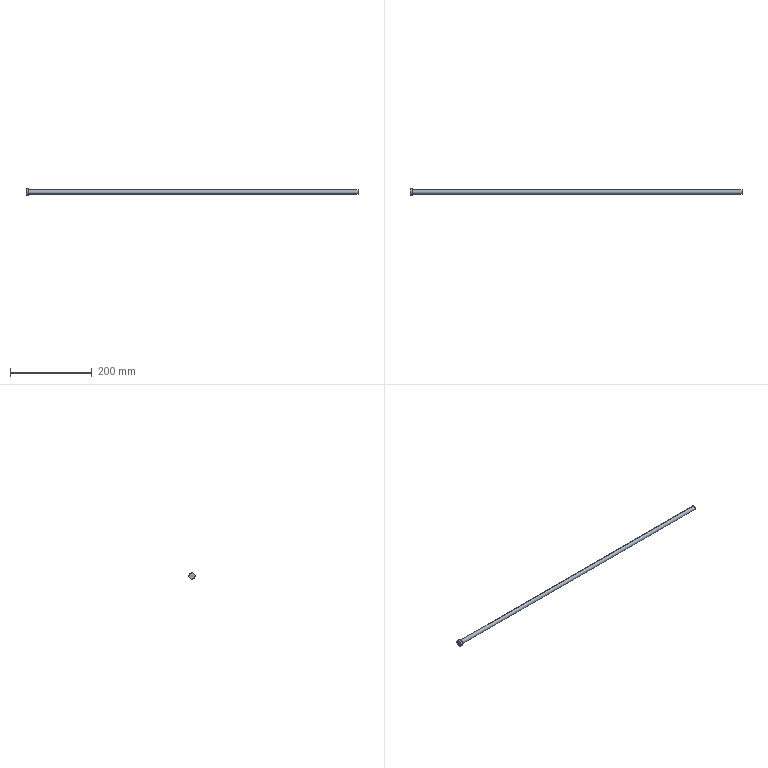Component | SolidWorks | SupportFastAxis-2 | 1 solid | 7 faces | box 811 x 15 x 15 mm | volume 64187 mm3 | cylinder 4 | plane 3 | commonest cylinder face diameters 15 x2 10 x2
build123d program:
from build123d import *

# Parameters (mm, degrees)
SKETCH1_R           = 5
BOSS_EXTRUDE1_DEPTH = 806
SKETCH2_R           = 7.5
BOSS_EXTRUDE2_DEPTH = 5


with BuildPart() as part:
    # Sketch1 → Boss-Extrude1 (new body)
    with BuildSketch(Plane.XY):
        with Locations((90, -65)):
            Circle(SKETCH1_R)
    extrude(amount=-BOSS_EXTRUDE1_DEPTH)

    # Sketch2 → Boss-Extrude2 (add)
    with BuildSketch(Plane.XY):
        with Locations((90, -65)):
            Circle(SKETCH2_R)
    extrude(amount=BOSS_EXTRUDE2_DEPTH)


solid = part.part

# Placed as in the assembly
solid = solid.moved(Location((-400, 155, -25), (0, -90, 0)))
STEP:
#1=COLOUR_RGB('',0.7922,0.8196,0.9333);
#2=FILL_AREA_STYLE_COLOUR('',#1);
#3=FILL_AREA_STYLE('',(#2));
#4=SURFACE_STYLE_FILL_AREA(#3);
#5=SURFACE_SIDE_STYLE('',(#4));
#6=SURFACE_STYLE_USAGE(.BOTH.,#5);
#7=PRESENTATION_STYLE_ASSIGNMENT((#6));
#8=CARTESIAN_POINT('',(-15.945,3.448,2.279));
#9=VERTEX_POINT('',#8);
#10=CARTESIAN_POINT('',(-15.945,3.638,2.839));
#11=VERTEX_POINT('',#10);
#12=CARTESIAN_POINT('',(-15.945,3.543,2.559));
#13=DIRECTION('',(-1.,0.,0.));
#14=DIRECTION('',(0.,-0.3218,-0.9468));
#15=AXIS2_PLACEMENT_3D('',#12,#13,#14);
#16=CIRCLE('',#15,0.2953);
#17=EDGE_CURVE('',#9,#11,#16,.T.);
#18=ORIENTED_EDGE('',*,*,#17,.F.);
#19=CARTESIAN_POINT('',(-15.748,3.448,2.279));
#20=VERTEX_POINT('',#19);
#21=CARTESIAN_POINT('',(-15.945,3.448,2.279));
#22=DIRECTION('',(1.,0.,0.));
#23=VECTOR('',#22,39.37);
#24=LINE('',#21,#23);
#25=EDGE_CURVE('',#9,#20,#24,.T.);
#26=ORIENTED_EDGE('',*,*,#25,.T.);
#27=CARTESIAN_POINT('',(-15.748,3.638,2.839));
#28=VERTEX_POINT('',#27);
#29=CARTESIAN_POINT('',(-15.748,3.543,2.559));
#30=DIRECTION('',(-1.,0.,0.));
#31=DIRECTION('',(0.,-0.3218,-0.9468));
#32=AXIS2_PLACEMENT_3D('',#29,#30,#31);
#33=CIRCLE('',#32,0.2953);
#34=EDGE_CURVE('',#20,#28,#33,.T.);
#35=ORIENTED_EDGE('',*,*,#34,.T.);
#36=CARTESIAN_POINT('',(-15.945,3.638,2.839));
#37=DIRECTION('',(1.,0.,0.));
#38=VECTOR('',#37,39.37);
#39=LINE('',#36,#38);
#40=EDGE_CURVE('',#11,#28,#39,.T.);
#41=ORIENTED_EDGE('',*,*,#40,.F.);
#42=EDGE_LOOP('',(#18,#26,#35,#41));
#43=FACE_OUTER_BOUND('',#42,.T.);
#44=CARTESIAN_POINT('',(-15.945,3.543,2.559));
#45=DIRECTION('',(1.,0.,0.));
#46=DIRECTION('',(0.,0.3218,0.9468));
#47=AXIS2_PLACEMENT_3D('',#44,#45,#46);
#48=CYLINDRICAL_SURFACE('',#47,0.2953);
#49=ADVANCED_FACE('',(#43),#48,.T.);
#50=CARTESIAN_POINT('',(15.984,3.48,2.373));
#51=VERTEX_POINT('',#50);
#52=CARTESIAN_POINT('',(15.984,3.607,2.745));
#53=VERTEX_POINT('',#52);
#54=CARTESIAN_POINT('',(15.984,3.543,2.559));
#55=DIRECTION('',(-1.,0.,0.));
#56=DIRECTION('',(0.,-0.3218,-0.9468));
#57=AXIS2_PLACEMENT_3D('',#54,#55,#56);
#58=CIRCLE('',#57,0.1969);
#59=EDGE_CURVE('',#51,#53,#58,.T.);
#60=ORIENTED_EDGE('',*,*,#59,.T.);
#61=CARTESIAN_POINT('',(-15.748,3.607,2.745));
#62=VERTEX_POINT('',#61);
#63=CARTESIAN_POINT('',(15.984,3.607,2.745));
#64=DIRECTION('',(-1.,0.,0.));
#65=VECTOR('',#64,39.37);
#66=LINE('',#63,#65);
#67=EDGE_CURVE('',#53,#62,#66,.T.);
#68=ORIENTED_EDGE('',*,*,#67,.T.);
#69=CARTESIAN_POINT('',(-15.748,3.48,2.373));
#70=VERTEX_POINT('',#69);
#71=CARTESIAN_POINT('',(-15.748,3.543,2.559));
#72=DIRECTION('',(-1.,0.,0.));
#73=DIRECTION('',(0.,-0.3218,-0.9468));
#74=AXIS2_PLACEMENT_3D('',#71,#72,#73);
#75=CIRCLE('',#74,0.1969);
#76=EDGE_CURVE('',#70,#62,#75,.T.);
#77=ORIENTED_EDGE('',*,*,#76,.F.);
#78=CARTESIAN_POINT('',(15.984,3.48,2.373));
#79=DIRECTION('',(-1.,0.,0.));
#80=VECTOR('',#79,39.37);
#81=LINE('',#78,#80);
#82=EDGE_CURVE('',#51,#70,#81,.T.);
#83=ORIENTED_EDGE('',*,*,#82,.F.);
#84=EDGE_LOOP('',(#60,#68,#77,#83));
#85=FACE_OUTER_BOUND('',#84,.T.);
#86=CARTESIAN_POINT('',(15.984,3.543,2.559));
#87=DIRECTION('',(-1.,0.,0.));
#88=DIRECTION('',(0.,-0.3218,-0.9468));
#89=AXIS2_PLACEMENT_3D('',#86,#87,#88);
#90=CYLINDRICAL_SURFACE('',#89,0.1969);
#91=ADVANCED_FACE('',(#85),#90,.T.);
#92=ORIENTED_EDGE('',*,*,#67,.F.);
#93=CARTESIAN_POINT('',(15.984,3.543,2.559));
#94=DIRECTION('',(-1.,0.,0.));
#95=DIRECTION('',(0.,-0.3218,-0.9468));
#96=AXIS2_PLACEMENT_3D('',#93,#94,#95);
#97=CIRCLE('',#96,0.1969);
#98=EDGE_CURVE('',#53,#51,#97,.T.);
#99=ORIENTED_EDGE('',*,*,#98,.T.);
#100=ORIENTED_EDGE('',*,*,#82,.T.);
#101=CARTESIAN_POINT('',(-15.748,3.543,2.559));
#102=DIRECTION('',(-1.,0.,0.));
#103=DIRECTION('',(0.,-0.3218,-0.9468));
#104=AXIS2_PLACEMENT_3D('',#101,#102,#103);
#105=CIRCLE('',#104,0.1969);
#106=EDGE_CURVE('',#62,#70,#105,.T.);
#107=ORIENTED_EDGE('',*,*,#106,.F.);
#108=EDGE_LOOP('',(#92,#99,#100,#107));
#109=FACE_OUTER_BOUND('',#108,.T.);
#110=CARTESIAN_POINT('',(15.984,3.543,2.559));
#111=DIRECTION('',(-1.,0.,0.));
#112=DIRECTION('',(0.,-0.3218,-0.9468));
#113=AXIS2_PLACEMENT_3D('',#110,#111,#112);
#114=CYLINDRICAL_SURFACE('',#113,0.1969);
#115=ADVANCED_FACE('',(#109),#114,.T.);
#116=ORIENTED_EDGE('',*,*,#59,.F.);
#117=ORIENTED_EDGE('',*,*,#98,.F.);
#118=EDGE_LOOP('',(#116,#117));
#119=FACE_OUTER_BOUND('',#118,.T.);
#120=CARTESIAN_POINT('',(15.984,3.543,2.559));
#121=DIRECTION('',(-1.,0.,0.));
#122=DIRECTION('',(0.,-0.3218,-0.9468));
#123=AXIS2_PLACEMENT_3D('',#120,#121,#122);
#124=PLANE('',#123);
#125=ADVANCED_FACE('',(#119),#124,.F.);
#126=ORIENTED_EDGE('',*,*,#25,.F.);
#127=CARTESIAN_POINT('',(-15.945,3.543,2.559));
#128=DIRECTION('',(-1.,0.,0.));
#129=DIRECTION('',(0.,-0.3218,-0.9468));
#130=AXIS2_PLACEMENT_3D('',#127,#128,#129);
#131=CIRCLE('',#130,0.2953);
#132=EDGE_CURVE('',#11,#9,#131,.T.);
#133=ORIENTED_EDGE('',*,*,#132,.F.);
#134=ORIENTED_EDGE('',*,*,#40,.T.);
#135=CARTESIAN_POINT('',(-15.748,3.543,2.559));
#136=DIRECTION('',(-1.,0.,0.));
#137=DIRECTION('',(0.,-0.3218,-0.9468));
#138=AXIS2_PLACEMENT_3D('',#135,#136,#137);
#139=CIRCLE('',#138,0.2953);
#140=EDGE_CURVE('',#28,#20,#139,.T.);
#141=ORIENTED_EDGE('',*,*,#140,.T.);
#142=EDGE_LOOP('',(#126,#133,#134,#141));
#143=FACE_OUTER_BOUND('',#142,.T.);
#144=CARTESIAN_POINT('',(-15.945,3.543,2.559));
#145=DIRECTION('',(1.,0.,0.));
#146=DIRECTION('',(0.,0.3218,0.9468));
#147=AXIS2_PLACEMENT_3D('',#144,#145,#146);
#148=CYLINDRICAL_SURFACE('',#147,0.2953);
#149=ADVANCED_FACE('',(#143),#148,.T.);
#150=ORIENTED_EDGE('',*,*,#132,.T.);
#151=ORIENTED_EDGE('',*,*,#17,.T.);
#152=EDGE_LOOP('',(#150,#151));
#153=FACE_OUTER_BOUND('',#152,.T.);
#154=CARTESIAN_POINT('',(-15.945,3.543,2.559));
#155=DIRECTION('',(-1.,0.,0.));
#156=DIRECTION('',(0.,-0.3218,-0.9468));
#157=AXIS2_PLACEMENT_3D('',#154,#155,#156);
#158=PLANE('',#157);
#159=ADVANCED_FACE('',(#153),#158,.T.);
#160=ORIENTED_EDGE('',*,*,#76,.T.);
#161=ORIENTED_EDGE('',*,*,#106,.T.);
#162=EDGE_LOOP('',(#160,#161));
#163=FACE_BOUND('',#162,.T.);
#164=ORIENTED_EDGE('',*,*,#140,.F.);
#165=ORIENTED_EDGE('',*,*,#34,.F.);
#166=EDGE_LOOP('',(#164,#165));
#167=FACE_OUTER_BOUND('',#166,.T.);
#168=CARTESIAN_POINT('',(-15.748,3.543,2.559));
#169=DIRECTION('',(-1.,0.,0.));
#170=DIRECTION('',(0.,-0.3218,-0.9468));
#171=AXIS2_PLACEMENT_3D('',#168,#169,#170);
#172=PLANE('',#171);
#173=ADVANCED_FACE('',(#163,#167),#172,.F.);
#174=CLOSED_SHELL('',(#49,#91,#115,#125,#149,#159,#173));
#175=MANIFOLD_SOLID_BREP('',#174);
#176=STYLED_ITEM('',(#7),#175);
#177=(LENGTH_UNIT()NAMED_UNIT(*)SI_UNIT($,.METRE.));
#178=LENGTH_MEASURE_WITH_UNIT(LENGTH_MEASURE(0.0254),#177);
#179=DIMENSIONAL_EXPONENTS(1.,0.,0.,0.,0.,0.,0.);
#180=(CONVERSION_BASED_UNIT('',#178)LENGTH_UNIT()NAMED_UNIT(#179));
#181=UNCERTAINTY_MEASURE_WITH_UNIT(LENGTH_MEASURE(0.00001),#180,'','');
#182=(NAMED_UNIT(*)PLANE_ANGLE_UNIT()SI_UNIT($,.RADIAN.));
#183=(NAMED_UNIT(*)SI_UNIT($,.STERADIAN.)SOLID_ANGLE_UNIT());
#184=(GEOMETRIC_REPRESENTATION_CONTEXT(3)GLOBAL_UNCERTAINTY_ASSIGNED_CONTEXT((#181))GLOBAL_UNIT_ASSIGNED_CONTEXT((#180,#182,#183))REPRESENTATION_CONTEXT('',''));
#185=MECHANICAL_DESIGN_GEOMETRIC_PRESENTATION_REPRESENTATION('',(#176),#184);
#186=CARTESIAN_POINT('',(0.,0.,0.));
#187=DIRECTION('',(0.,0.,1.));
#188=DIRECTION('',(1.,0.,0.));
#189=AXIS2_PLACEMENT_3D('',#186,#187,#188);
#190=(LENGTH_UNIT()NAMED_UNIT(*)SI_UNIT($,.METRE.));
#191=LENGTH_MEASURE_WITH_UNIT(LENGTH_MEASURE(0.0254),#190);
#192=DIMENSIONAL_EXPONENTS(1.,0.,0.,0.,0.,0.,0.);
#193=(CONVERSION_BASED_UNIT('',#191)LENGTH_UNIT()NAMED_UNIT(#192));
#194=UNCERTAINTY_MEASURE_WITH_UNIT(LENGTH_MEASURE(0.00001),#193,'','');
#195=(NAMED_UNIT(*)PLANE_ANGLE_UNIT()SI_UNIT($,.RADIAN.));
#196=(NAMED_UNIT(*)SI_UNIT($,.STERADIAN.)SOLID_ANGLE_UNIT());
#197=(GEOMETRIC_REPRESENTATION_CONTEXT(3)GLOBAL_UNCERTAINTY_ASSIGNED_CONTEXT((#194))GLOBAL_UNIT_ASSIGNED_CONTEXT((#193,#195,#196))REPRESENTATION_CONTEXT('',''));
#198=ADVANCED_BREP_SHAPE_REPRESENTATION('',(#175,#189),#197);
#199=PRESENTATION_LAYER_ASSIGNMENT('','',(#176));